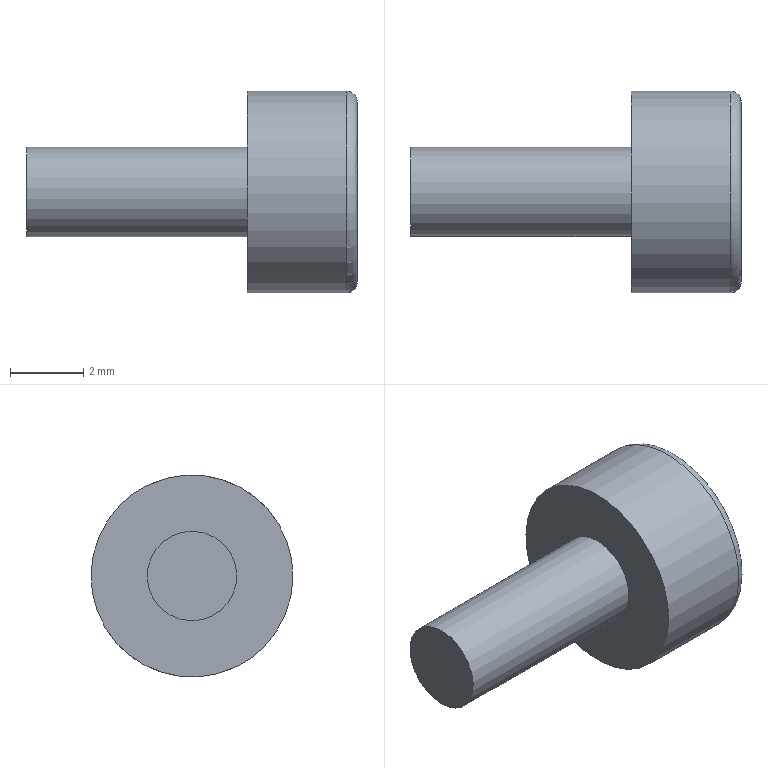Component | NX | GB70_2-M3X6_17 | 1 solid | 25 faces | volume 88 mm3 | plane 15 | cone 7 | cylinder 2 | torus 1 | commonest cylinder face diameters 5.5 x1 2.44 x1